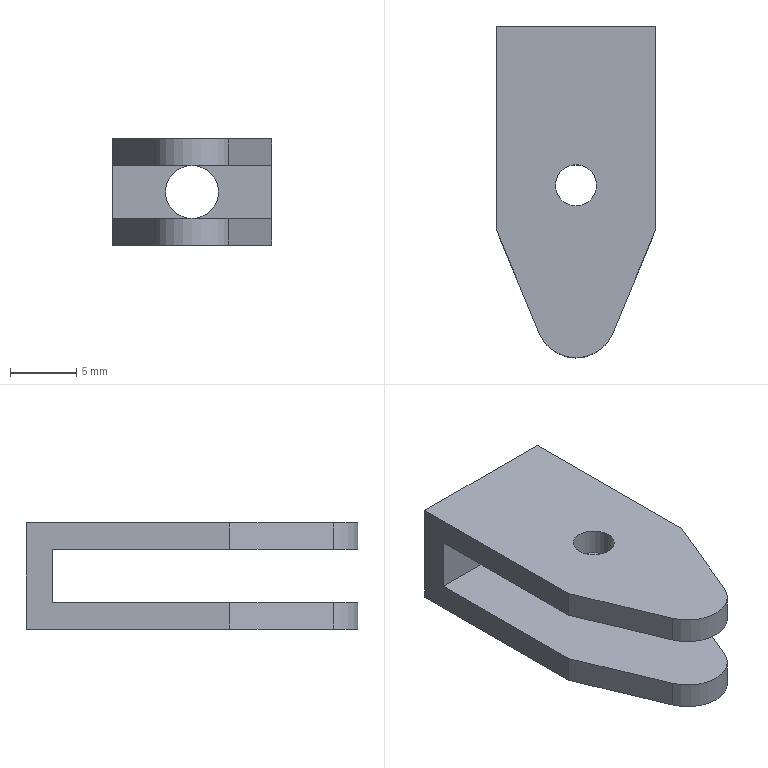Component | NX | 02 | 1 solid | 18 faces | volume 1081 mm3 | plane 13 | cylinder 5 | commonest cylinder face diameters 6 x2 3.1 x2 4 x1